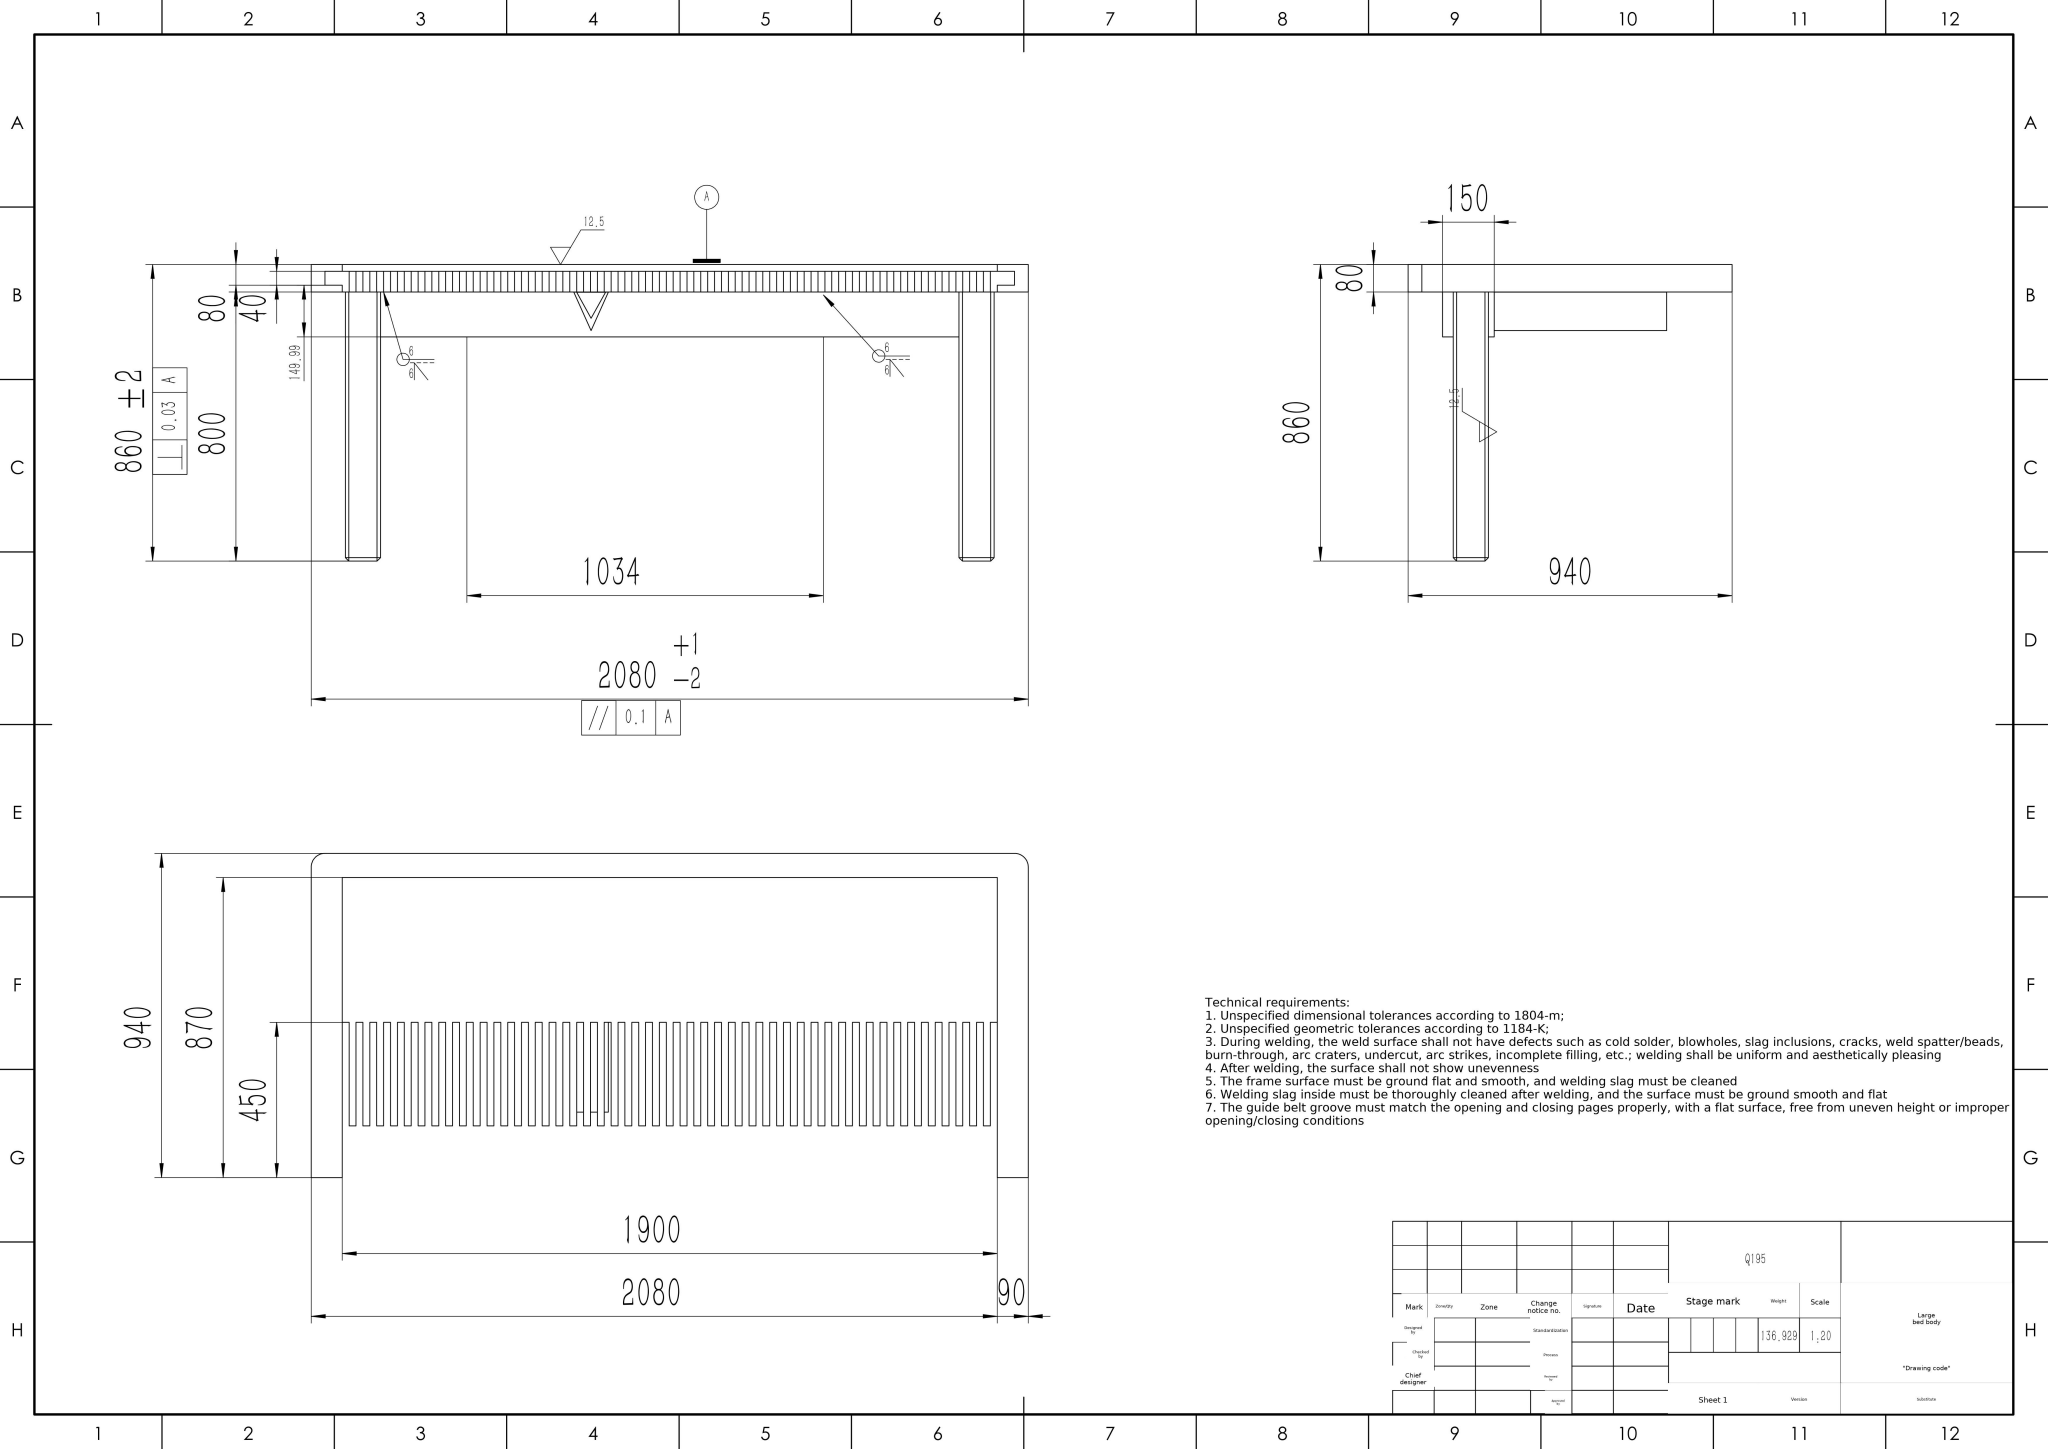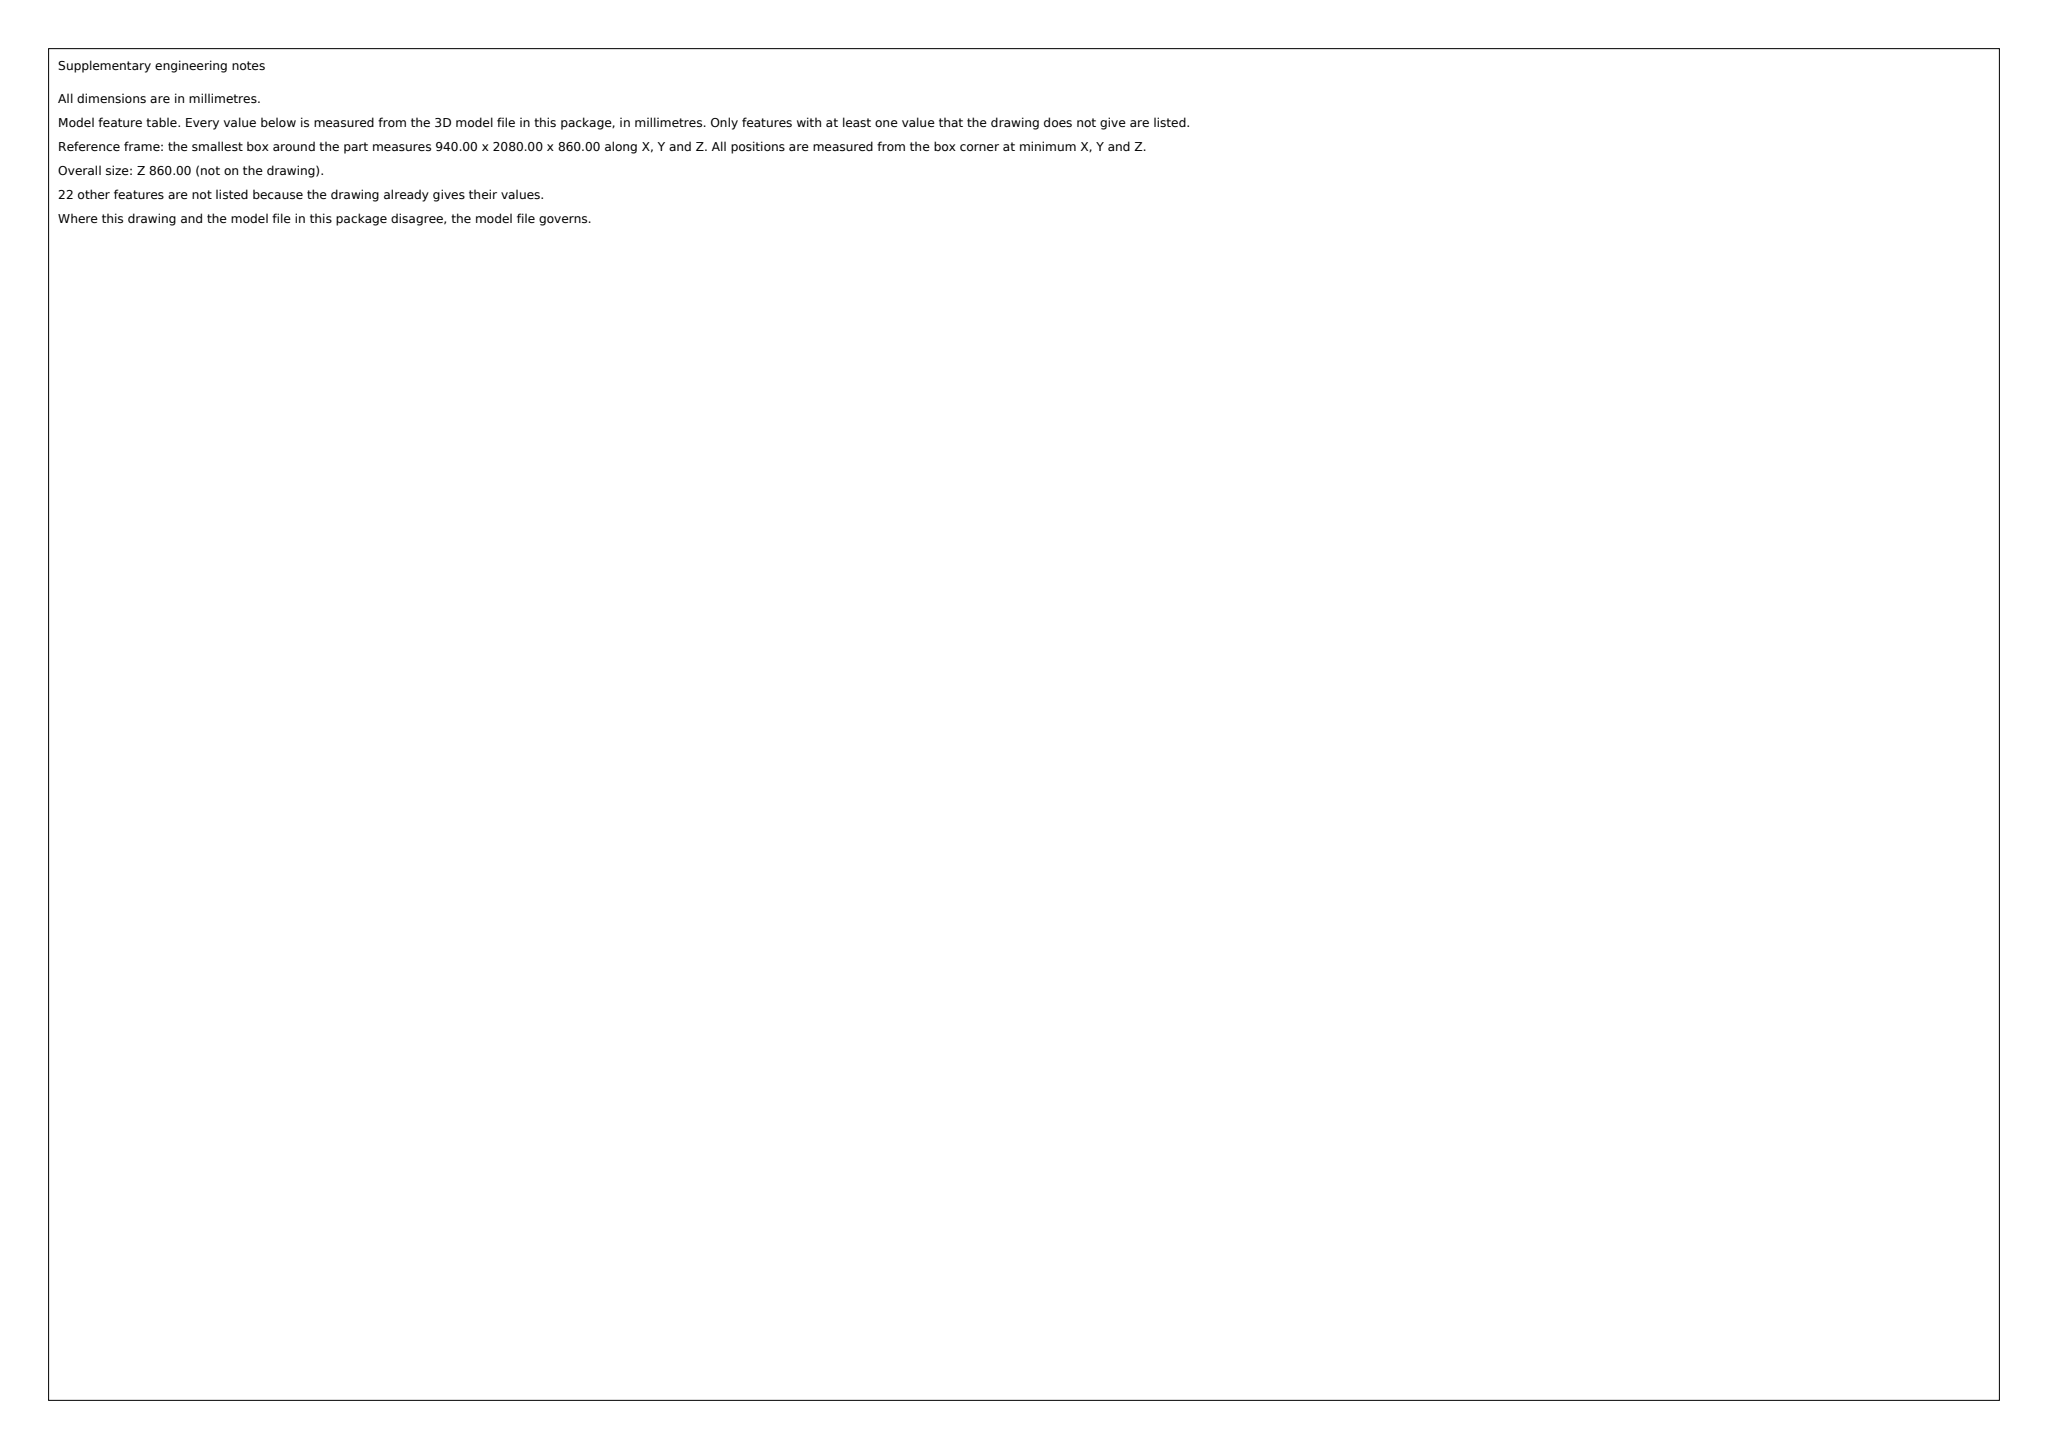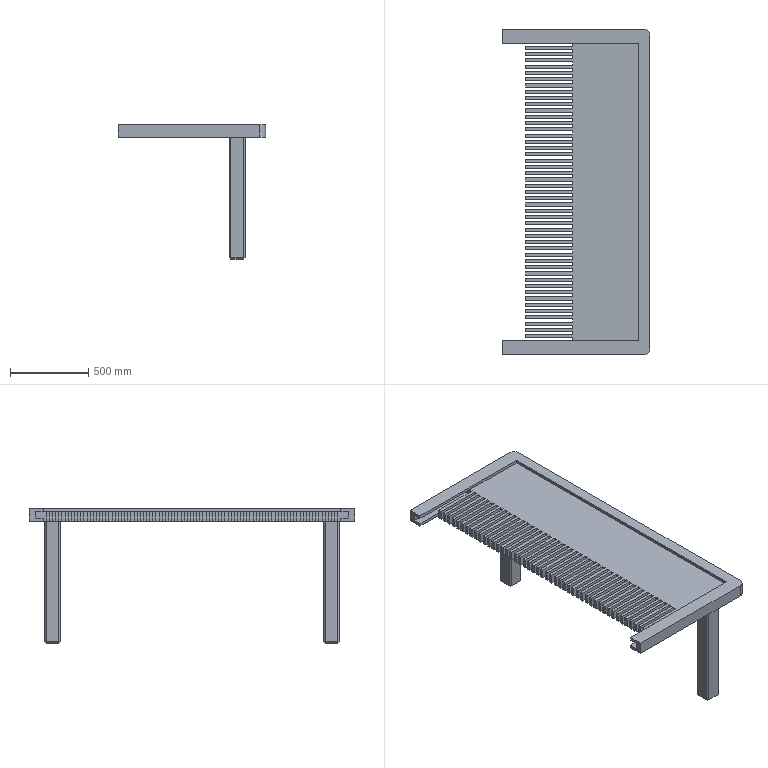Part | SolidWorks | mm | material Q195 | 1 solid | 268 faces | box 940 x 2080 x 860 mm | volume 102998755 mm3 | plane 242 | cylinder 18 | cone 8 | commonest cylinder face diameters 8.8 x16 80 x2